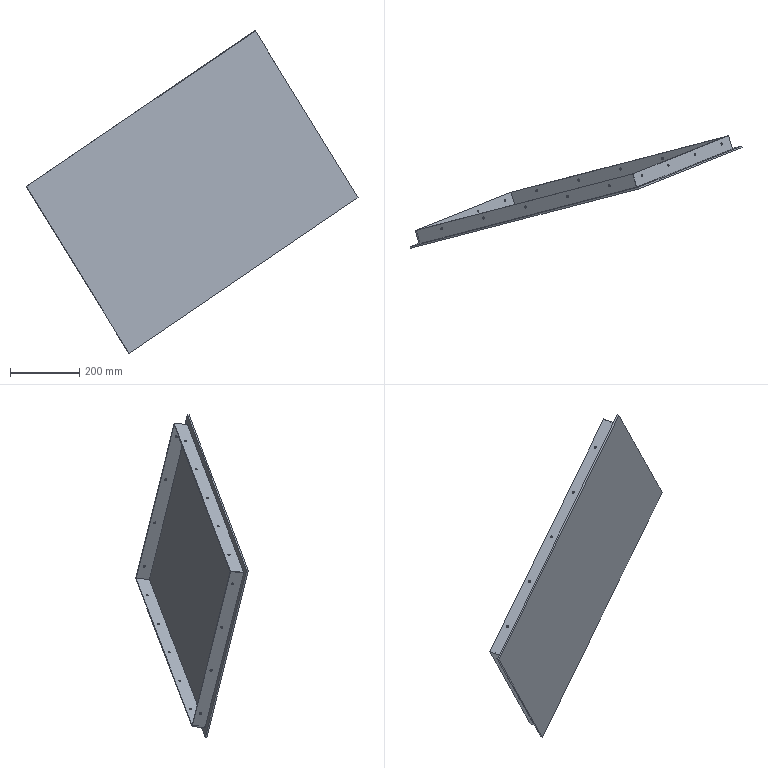Component | SolidWorks | CrusherFrameTopCover-1 | 1 solid | 52 faces | box 962.05 x 326.17 x 934.23 mm | volume 2691833 mm3 | cylinder 36 | plane 16 | commonest cylinder face diameters 6 x36
build123d program:
from build123d import *

# Parameters (mm, degrees)
SKETCH1_W          = 820
SKETCH1_H          = 580
EXTRUDE1_DEPTH     = 45
SKETCH2_W          = 820
SKETCH2_H          = 580
SKETCH2_W_2        = 780
SKETCH2_H_2        = 540
SKETCH2_W_3        = 774
SKETCH2_H_3        = 534
CUT_EXTRUDE1_DEPTH = 40
SKETCH3_R          = 3
CUT_EXTRUDE2_DEPTH = 990.154
SKETCH4_R          = 3
CUT_EXTRUDE3_DEPTH = 994.994
LPATTERN1_COUNT    = 5
LPATTERN1_PITCH    = 150
LPATTERN2_COUNT    = 4
LPATTERN2_PITCH    = 150


with BuildPart() as part:
    # Sketch1 → Extrude1 (new body)
    with BuildSketch(Plane.XY):
        with Locations((410, 290)):
            Rectangle(SKETCH1_W, SKETCH1_H)
    extrude(amount=EXTRUDE1_DEPTH)

    # Sketch2 → Cut-Extrude1 (cut)
    # profile 1 of 2: a face of its own
    with BuildSketch(Plane.XY.offset(45)):
        with Locations((410, 290)):
            Rectangle(SKETCH2_W, SKETCH2_H)
        with Locations((410, 290)):
            Rectangle(SKETCH2_W_2, SKETCH2_H_2, mode=Mode.SUBTRACT)
    # profile 2 of 2: a face of its own
    with BuildSketch(Plane.XY.offset(45)):
        with Locations((410, 290)):
            Rectangle(SKETCH2_W_3, SKETCH2_H_3)
    extrude(amount=-CUT_EXTRUDE1_DEPTH, mode=Mode.SUBTRACT)

    # Sketch3 → Cut-Extrude2 (cut, through all)
    with BuildSketch(Plane(origin=(800, 0, 0), x_dir=(0, 0, -1), z_dir=(1, 0, 0))):
        with Locations(Location((-30, 513, 0), (0, 0, 90))):
            Circle(SKETCH3_R)
    cut_extrude2 = extrude(amount=-CUT_EXTRUDE2_DEPTH, mode=Mode.SUBTRACT)

    # Sketch4 → Cut-Extrude3 (cut, through all)
    with BuildSketch(Plane(origin=(0, 560, 0), x_dir=(1, 0, 0), z_dir=(0, 1, 0))):
        with Locations((710, -30)):
            Circle(SKETCH4_R)
    cut_extrude3 = extrude(amount=-CUT_EXTRUDE3_DEPTH, mode=Mode.SUBTRACT)

    # LPattern1: Cut-Extrude3 ×5
    with Locations(*[(-i * LPATTERN1_PITCH, 0, 0) for i in range(1, LPATTERN1_COUNT)]):
        add(cut_extrude3, mode=Mode.SUBTRACT)

    # LPattern2: Cut-Extrude2 ×4
    with Locations(*[(0, -i * LPATTERN2_PITCH, 0) for i in range(1, LPATTERN2_COUNT)]):
        add(cut_extrude2, mode=Mode.SUBTRACT)


solid = part.part

# Placed as in the assembly
solid = solid.moved(Location((-395.48, -549.638, -258.54), (-86.429, -16.737, -32.369)))